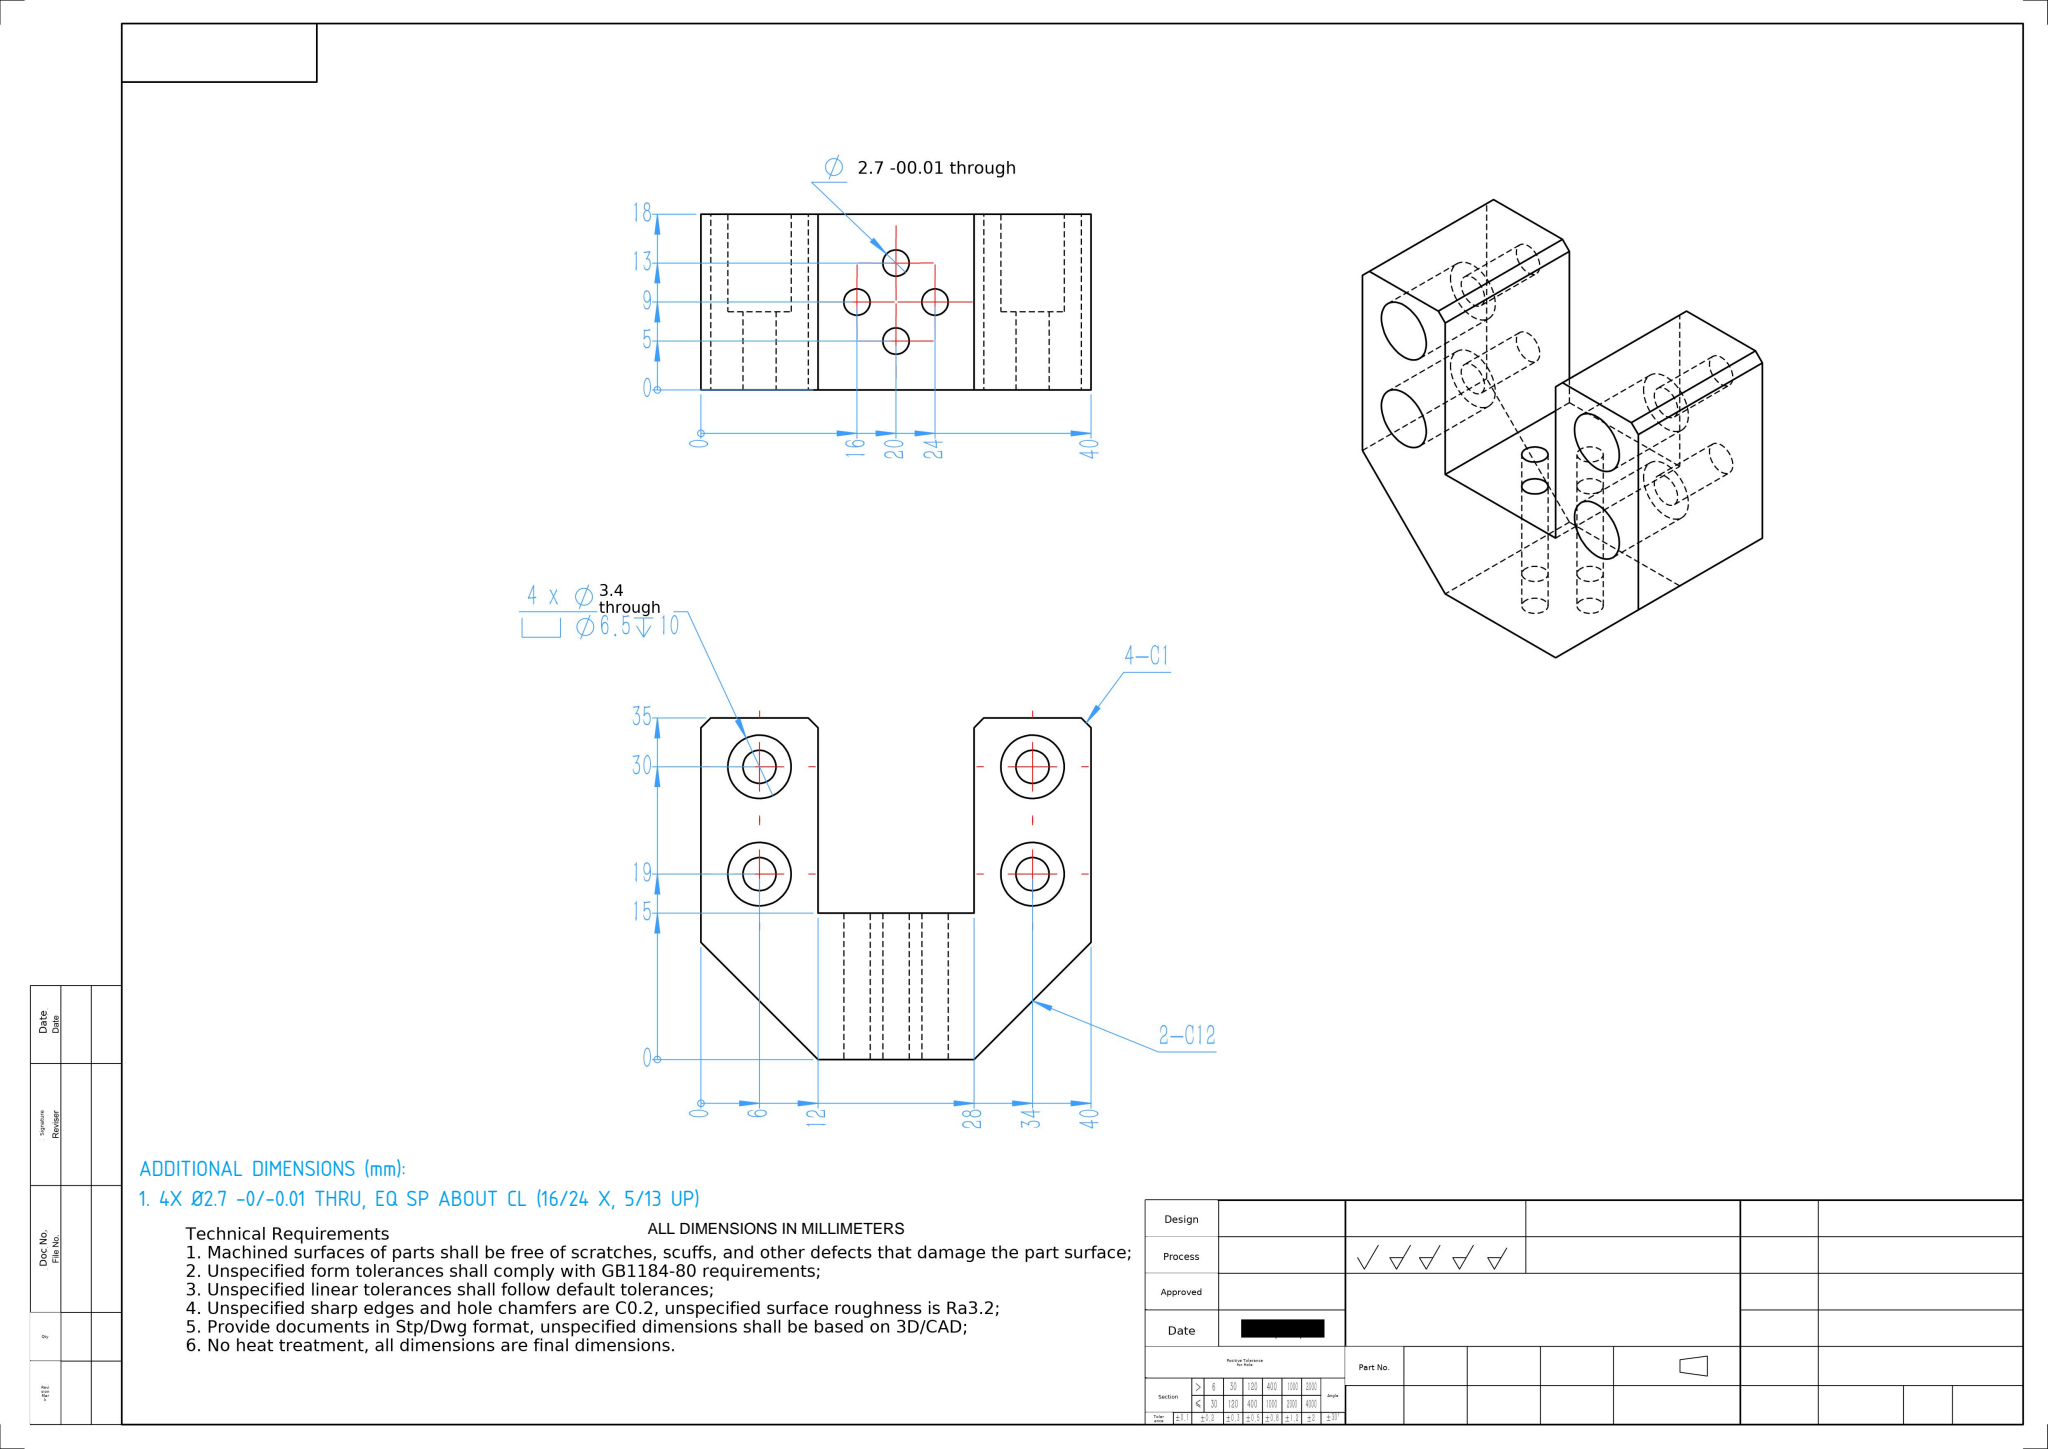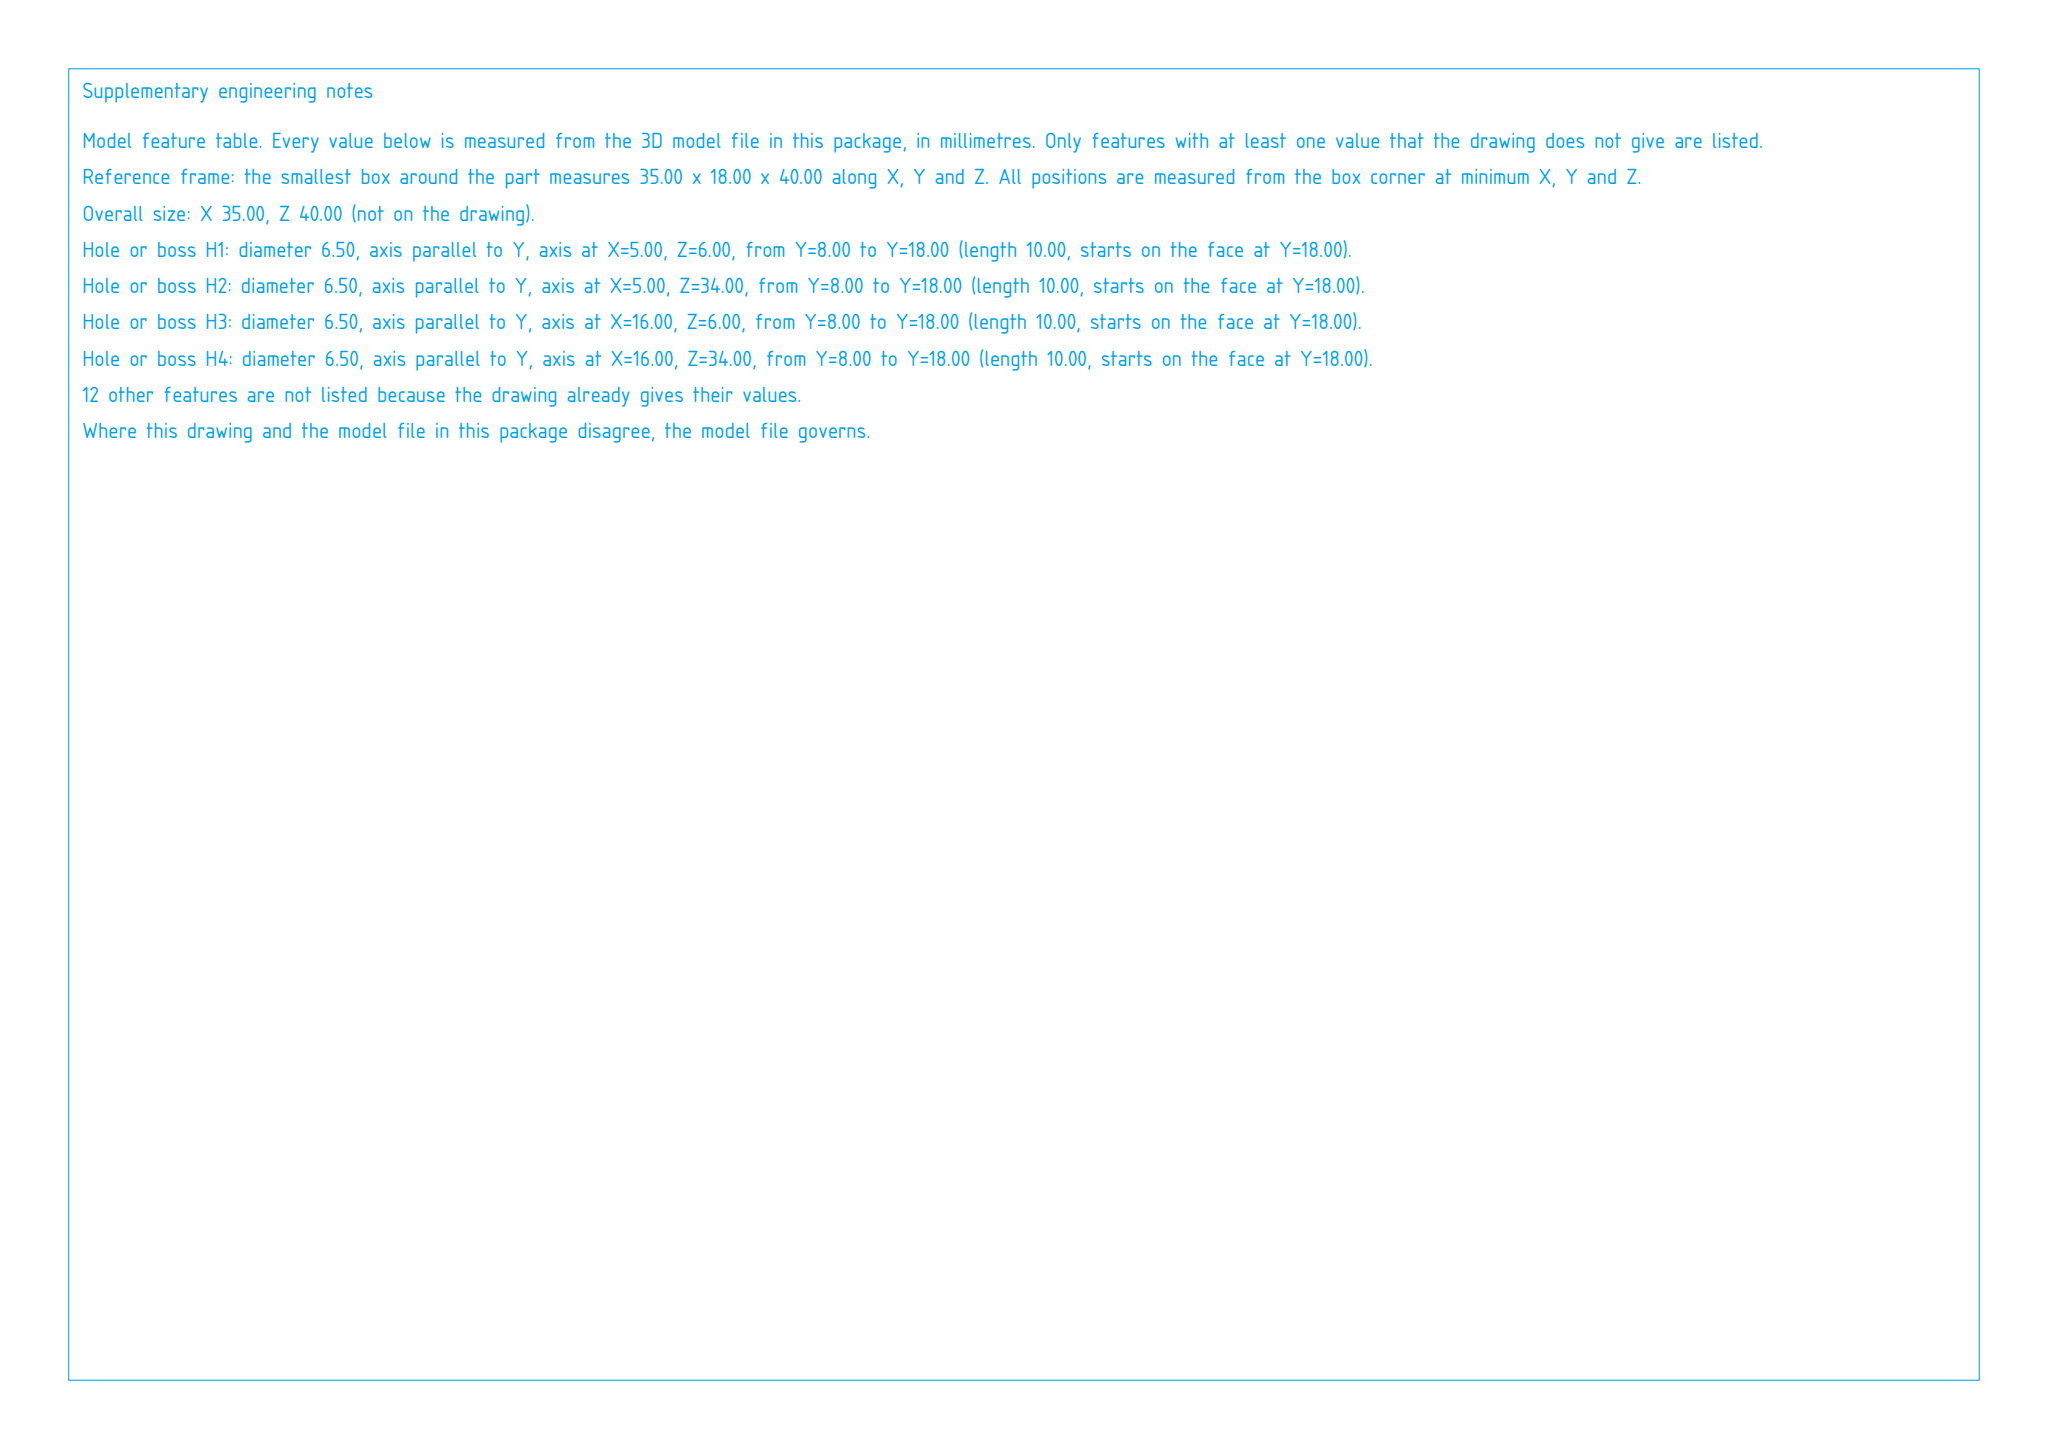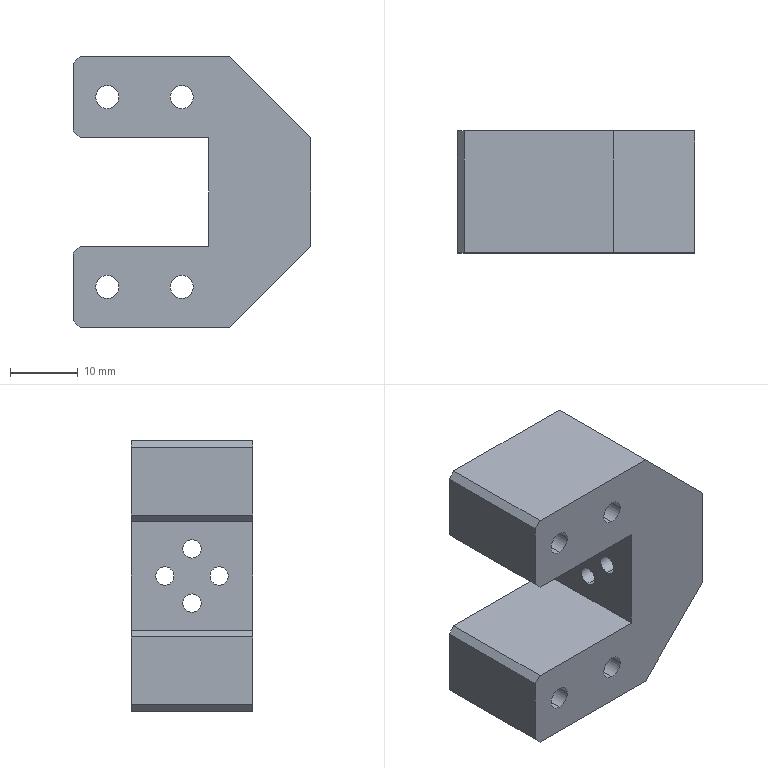Part | SolidWorks | mm | 1 solid | 44 faces | box 35 x 18 x 40 mm | volume 14851 mm3 | cylinder 24 | plane 20 | commonest cylinder face diameters 6.5 x8 3.4 x8 2.7 x8
build123d program:
from build123d import *

# Parameters (mm, degrees)
SKETCH1_W                                       = 35
SKETCH1_H                                       = 40
BOSS_EXTRUDE1_DEPTH                             = 40
SKETCH2_W                                       = 35
SKETCH2_H                                       = 22
CUT_EXTRUDE1_DEPTH                              = 49.023
SKETCH3_W                                       = 20
SKETCH3_H                                       = 16
CUT_EXTRUDE2_DEPTH                              = 18
SKETCH4_R                                       = 1.35
CUT_EXTRUDE3_DEPTH                              = 49.99
CHAMFER1_SIZE                                   = 1
CHAMFER2_SIZE                                   = 12
M3_HEX_SOCKET_HEAD_CAP_SCREW_CBORE1_D           = 3.4
M3_HEX_SOCKET_HEAD_CAP_SCREW_CBORE1_CBORE_D     = 6.5
M3_HEX_SOCKET_HEAD_CAP_SCREW_CBORE1_CBORE_DEPTH = 10


with BuildPart() as part:
    # Sketch1 → Boss-Extrude1 (new body)
    with BuildSketch(Plane.XY):
        Rectangle(SKETCH1_W, SKETCH1_H)
    extrude(amount=BOSS_EXTRUDE1_DEPTH)

    # Sketch2 → Cut-Extrude1 (cut, through all)
    with BuildSketch(Plane.XY.offset(40)):
        with Locations((0, -9)):
            Rectangle(SKETCH2_W, SKETCH2_H)
    extrude(amount=-CUT_EXTRUDE1_DEPTH, mode=Mode.SUBTRACT)

    # Sketch3 → Cut-Extrude2 (cut)
    with BuildSketch(Plane(origin=(0, 20, 0), x_dir=(1, 0, 0), z_dir=(0, 1, 0))):
        with Locations((-7.5, -20)):
            Rectangle(SKETCH3_W, SKETCH3_H)
    extrude(amount=-CUT_EXTRUDE2_DEPTH, mode=Mode.SUBTRACT)

    # Sketch4 → Cut-Extrude3 (cut, through all)
    with BuildSketch(Plane.ZY.offset(-2.5)):
        with Locations((20, 15)):
            Circle(SKETCH4_R)
        with Locations((24, 11)):
            Circle(SKETCH4_R)
        with Locations((16, 11)):
            Circle(SKETCH4_R)
        with Locations((20, 7)):
            Circle(SKETCH4_R)
    extrude(amount=-CUT_EXTRUDE3_DEPTH, mode=Mode.SUBTRACT)

    # Chamfer1
    chamfer1_edges = [part.edges().sort_by_distance(p)[0] for p in [
        (-17.5, 11, 40),
        (-17.5, 11, 28),
        (-17.5, 11, 12),
        (-17.5, 11, 0),
    ]]
    chamfer(chamfer1_edges, length=CHAMFER1_SIZE)

    # Chamfer2
    chamfer2_edges = [part.edges().sort_by_distance(p)[0] for p in [
        (17.5, 11, 0),
        (17.5, 11, 40),
    ]]
    chamfer(chamfer2_edges, length=CHAMFER2_SIZE)

    # M3 Hex Socket Head Cap Screw CBORE1 (through all)
    with Locations(Plane(origin=(0, 20, 0), x_dir=(1, 0, 0), z_dir=(0, 1, 0))):
        with Locations((-12.5, -34), (-1.5, -34), (-1.5, -6), (-12.5, -6)):
            CounterBoreHole(M3_HEX_SOCKET_HEAD_CAP_SCREW_CBORE1_D / 2, M3_HEX_SOCKET_HEAD_CAP_SCREW_CBORE1_CBORE_D / 2, M3_HEX_SOCKET_HEAD_CAP_SCREW_CBORE1_CBORE_DEPTH)


solid = part.part